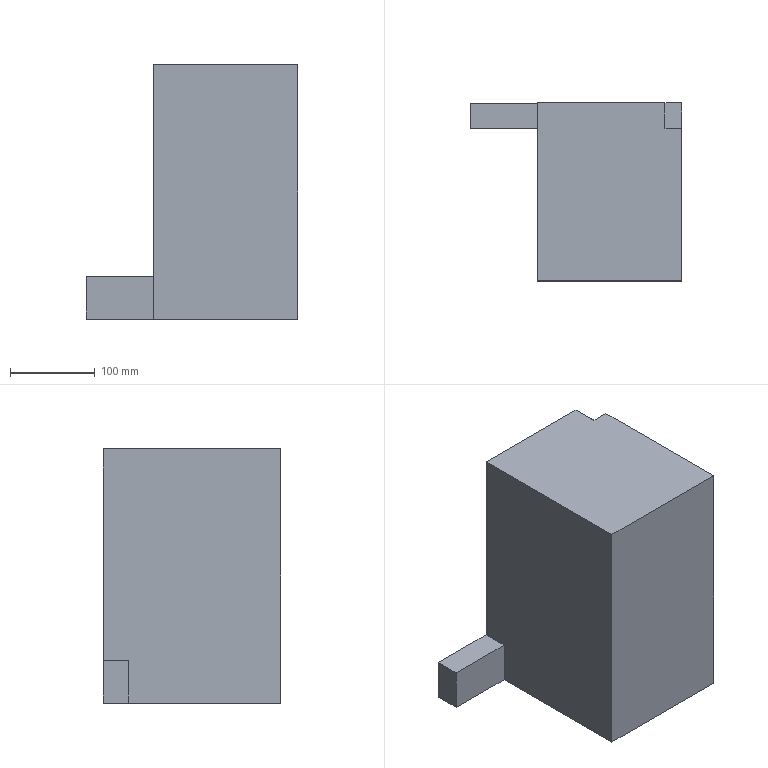Component | SolidWorks | -3[2]-1 | 1 solid | 14 faces | box 250 x 210 x 300 mm | volume 10806823 mm3 | plane 12 | cylinder 2 | commonest cylinder face diameters 27 x2
STEP:
#1=CARTESIAN_POINT('',(19.685,-89.764,-4.39));
#2=VERTEX_POINT('',#1);
#3=CARTESIAN_POINT('',(19.685,-89.764,-5.453));
#4=VERTEX_POINT('',#3);
#5=CARTESIAN_POINT('',(19.685,-89.764,-4.921));
#6=DIRECTION('',(0.,-1.,0.));
#7=DIRECTION('',(0.,0.,1.));
#8=AXIS2_PLACEMENT_3D('',#5,#6,#7);
#9=CIRCLE('',#8,0.5315);
#10=EDGE_CURVE('',#2,#4,#9,.T.);
#11=ORIENTED_EDGE('',*,*,#10,.T.);
#12=CARTESIAN_POINT('',(19.685,-88.583,-5.453));
#13=VERTEX_POINT('',#12);
#14=CARTESIAN_POINT('',(19.685,-89.764,-5.453));
#15=DIRECTION('',(0.,1.,0.));
#16=VECTOR('',#15,39.37);
#17=LINE('',#14,#16);
#18=EDGE_CURVE('',#4,#13,#17,.T.);
#19=ORIENTED_EDGE('',*,*,#18,.T.);
#20=CARTESIAN_POINT('',(19.685,-88.583,-4.39));
#21=VERTEX_POINT('',#20);
#22=CARTESIAN_POINT('',(19.685,-88.583,-4.921));
#23=DIRECTION('',(0.,-1.,0.));
#24=DIRECTION('',(0.,0.,1.));
#25=AXIS2_PLACEMENT_3D('',#22,#23,#24);
#26=CIRCLE('',#25,0.5315);
#27=EDGE_CURVE('',#21,#13,#26,.T.);
#28=ORIENTED_EDGE('',*,*,#27,.F.);
#29=CARTESIAN_POINT('',(19.685,-89.764,-4.39));
#30=DIRECTION('',(0.,1.,0.));
#31=VECTOR('',#30,39.37);
#32=LINE('',#29,#31);
#33=EDGE_CURVE('',#2,#21,#32,.T.);
#34=ORIENTED_EDGE('',*,*,#33,.F.);
#35=EDGE_LOOP('',(#11,#19,#28,#34));
#36=FACE_OUTER_BOUND('',#35,.T.);
#37=CARTESIAN_POINT('',(19.685,-89.764,-4.921));
#38=DIRECTION('',(0.,1.,0.));
#39=DIRECTION('',(0.,0.,-1.));
#40=AXIS2_PLACEMENT_3D('',#37,#38,#39);
#41=CYLINDRICAL_SURFACE('',#40,0.5315);
#42=ADVANCED_FACE('',(#36),#41,.F.);
#43=CARTESIAN_POINT('',(14.961,-89.764,-6.89));
#44=VERTEX_POINT('',#43);
#45=CARTESIAN_POINT('',(14.961,-89.764,-8.858));
#46=VERTEX_POINT('',#45);
#47=CARTESIAN_POINT('',(14.961,-89.764,2.953));
#48=DIRECTION('',(0.,0.,-1.));
#49=VECTOR('',#48,39.37);
#50=LINE('',#47,#49);
#51=EDGE_CURVE('',#44,#46,#50,.T.);
#52=ORIENTED_EDGE('',*,*,#51,.F.);
#53=CARTESIAN_POINT('',(11.811,-89.764,-6.89));
#54=VERTEX_POINT('',#53);
#55=CARTESIAN_POINT('',(14.961,-89.764,-6.89));
#56=DIRECTION('',(-1.,0.,0.));
#57=VECTOR('',#56,39.37);
#58=LINE('',#55,#57);
#59=EDGE_CURVE('',#44,#54,#58,.T.);
#60=ORIENTED_EDGE('',*,*,#59,.T.);
#61=CARTESIAN_POINT('',(11.811,-89.764,-8.858));
#62=VERTEX_POINT('',#61);
#63=CARTESIAN_POINT('',(11.811,-89.764,-6.89));
#64=DIRECTION('',(0.,0.,-1.));
#65=VECTOR('',#64,39.37);
#66=LINE('',#63,#65);
#67=EDGE_CURVE('',#54,#62,#66,.T.);
#68=ORIENTED_EDGE('',*,*,#67,.T.);
#69=CARTESIAN_POINT('',(11.811,-89.764,-8.858));
#70=DIRECTION('',(1.,0.,0.));
#71=VECTOR('',#70,39.37);
#72=LINE('',#69,#71);
#73=EDGE_CURVE('',#62,#46,#72,.T.);
#74=ORIENTED_EDGE('',*,*,#73,.T.);
#75=EDGE_LOOP('',(#52,#60,#68,#74));
#76=FACE_OUTER_BOUND('',#75,.T.);
#77=CARTESIAN_POINT('',(11.811,-89.764,-8.858));
#78=DIRECTION('',(0.,-1.,0.));
#79=DIRECTION('',(0.,0.,1.));
#80=AXIS2_PLACEMENT_3D('',#77,#78,#79);
#81=PLANE('',#80);
#82=ADVANCED_FACE('',(#76),#81,.T.);
#83=CARTESIAN_POINT('',(11.811,-88.583,-6.89));
#84=VERTEX_POINT('',#83);
#85=CARTESIAN_POINT('',(11.811,-88.583,-8.858));
#86=VERTEX_POINT('',#85);
#87=CARTESIAN_POINT('',(11.811,-88.583,-6.89));
#88=DIRECTION('',(0.,0.,-1.));
#89=VECTOR('',#88,39.37);
#90=LINE('',#87,#89);
#91=EDGE_CURVE('',#84,#86,#90,.T.);
#92=ORIENTED_EDGE('',*,*,#91,.F.);
#93=CARTESIAN_POINT('',(14.961,-88.583,-6.89));
#94=VERTEX_POINT('',#93);
#95=CARTESIAN_POINT('',(14.961,-88.583,-6.89));
#96=DIRECTION('',(-1.,0.,0.));
#97=VECTOR('',#96,39.37);
#98=LINE('',#95,#97);
#99=EDGE_CURVE('',#94,#84,#98,.T.);
#100=ORIENTED_EDGE('',*,*,#99,.F.);
#101=CARTESIAN_POINT('',(14.961,-88.583,2.953));
#102=VERTEX_POINT('',#101);
#103=CARTESIAN_POINT('',(14.961,-88.583,2.953));
#104=DIRECTION('',(-0.,0.,-1.));
#105=VECTOR('',#104,39.37);
#106=LINE('',#103,#105);
#107=EDGE_CURVE('',#102,#94,#106,.T.);
#108=ORIENTED_EDGE('',*,*,#107,.F.);
#109=CARTESIAN_POINT('',(20.866,-88.583,2.953));
#110=VERTEX_POINT('',#109);
#111=CARTESIAN_POINT('',(20.866,-88.583,2.953));
#112=DIRECTION('',(-1.,0.,0.));
#113=VECTOR('',#112,39.37);
#114=LINE('',#111,#113);
#115=EDGE_CURVE('',#110,#102,#114,.T.);
#116=ORIENTED_EDGE('',*,*,#115,.F.);
#117=CARTESIAN_POINT('',(21.654,-88.583,2.165));
#118=VERTEX_POINT('',#117);
#119=CARTESIAN_POINT('',(21.654,-88.583,2.165));
#120=DIRECTION('',(-0.7071,0.,0.7071));
#121=VECTOR('',#120,39.37);
#122=LINE('',#119,#121);
#123=EDGE_CURVE('',#118,#110,#122,.T.);
#124=ORIENTED_EDGE('',*,*,#123,.F.);
#125=CARTESIAN_POINT('',(21.654,-88.583,-8.858));
#126=VERTEX_POINT('',#125);
#127=CARTESIAN_POINT('',(21.654,-88.583,-8.858));
#128=DIRECTION('',(0.,0.,1.));
#129=VECTOR('',#128,39.37);
#130=LINE('',#127,#129);
#131=EDGE_CURVE('',#126,#118,#130,.T.);
#132=ORIENTED_EDGE('',*,*,#131,.F.);
#133=CARTESIAN_POINT('',(11.811,-88.583,-8.858));
#134=DIRECTION('',(1.,0.,0.));
#135=VECTOR('',#134,39.37);
#136=LINE('',#133,#135);
#137=EDGE_CURVE('',#86,#126,#136,.T.);
#138=ORIENTED_EDGE('',*,*,#137,.F.);
#139=EDGE_LOOP('',(#92,#100,#108,#116,#124,#132,#138));
#140=FACE_OUTER_BOUND('',#139,.T.);
#141=ORIENTED_EDGE('',*,*,#27,.T.);
#142=CARTESIAN_POINT('',(19.685,-88.583,-4.921));
#143=DIRECTION('',(0.,-1.,0.));
#144=DIRECTION('',(0.,0.,1.));
#145=AXIS2_PLACEMENT_3D('',#142,#143,#144);
#146=CIRCLE('',#145,0.5315);
#147=EDGE_CURVE('',#13,#21,#146,.T.);
#148=ORIENTED_EDGE('',*,*,#147,.T.);
#149=EDGE_LOOP('',(#141,#148));
#150=FACE_BOUND('',#149,.T.);
#151=CARTESIAN_POINT('',(11.811,-88.583,-8.858));
#152=DIRECTION('',(0.,-1.,0.));
#153=DIRECTION('',(0.,0.,1.));
#154=AXIS2_PLACEMENT_3D('',#151,#152,#153);
#155=PLANE('',#154);
#156=ADVANCED_FACE('',(#140,#150),#155,.F.);
#157=ORIENTED_EDGE('',*,*,#91,.T.);
#158=CARTESIAN_POINT('',(11.811,-89.764,-8.858));
#159=DIRECTION('',(0.,1.,0.));
#160=VECTOR('',#159,39.37);
#161=LINE('',#158,#160);
#162=EDGE_CURVE('',#62,#86,#161,.T.);
#163=ORIENTED_EDGE('',*,*,#162,.F.);
#164=ORIENTED_EDGE('',*,*,#67,.F.);
#165=CARTESIAN_POINT('',(11.811,-89.764,-6.89));
#166=DIRECTION('',(0.,1.,0.));
#167=VECTOR('',#166,39.37);
#168=LINE('',#165,#167);
#169=EDGE_CURVE('',#54,#84,#168,.T.);
#170=ORIENTED_EDGE('',*,*,#169,.T.);
#171=EDGE_LOOP('',(#157,#163,#164,#170));
#172=FACE_OUTER_BOUND('',#171,.T.);
#173=CARTESIAN_POINT('',(11.811,-89.764,-6.89));
#174=DIRECTION('',(1.,0.,0.));
#175=DIRECTION('',(0.,0.,1.));
#176=AXIS2_PLACEMENT_3D('',#173,#174,#175);
#177=PLANE('',#176);
#178=ADVANCED_FACE('',(#172),#177,.F.);
#179=ORIENTED_EDGE('',*,*,#137,.T.);
#180=CARTESIAN_POINT('',(21.654,-96.85,-8.858));
#181=VERTEX_POINT('',#180);
#182=CARTESIAN_POINT('',(21.654,-89.764,-8.858));
#183=DIRECTION('',(0.,1.,0.));
#184=VECTOR('',#183,39.37);
#185=LINE('',#182,#184);
#186=EDGE_CURVE('',#181,#126,#185,.T.);
#187=ORIENTED_EDGE('',*,*,#186,.F.);
#188=CARTESIAN_POINT('',(14.961,-96.85,-8.858));
#189=VERTEX_POINT('',#188);
#190=CARTESIAN_POINT('',(14.961,-96.85,-8.858));
#191=DIRECTION('',(1.,0.,0.));
#192=VECTOR('',#191,39.37);
#193=LINE('',#190,#192);
#194=EDGE_CURVE('',#189,#181,#193,.T.);
#195=ORIENTED_EDGE('',*,*,#194,.F.);
#196=CARTESIAN_POINT('',(14.961,-96.85,-8.858));
#197=DIRECTION('',(0.,1.,0.));
#198=VECTOR('',#197,39.37);
#199=LINE('',#196,#198);
#200=EDGE_CURVE('',#189,#46,#199,.T.);
#201=ORIENTED_EDGE('',*,*,#200,.T.);
#202=ORIENTED_EDGE('',*,*,#73,.F.);
#203=ORIENTED_EDGE('',*,*,#162,.T.);
#204=EDGE_LOOP('',(#179,#187,#195,#201,#202,#203));
#205=FACE_OUTER_BOUND('',#204,.T.);
#206=CARTESIAN_POINT('',(11.811,-89.764,-8.858));
#207=DIRECTION('',(0.,0.,1.));
#208=DIRECTION('',(-1.,0.,0.));
#209=AXIS2_PLACEMENT_3D('',#206,#207,#208);
#210=PLANE('',#209);
#211=ADVANCED_FACE('',(#205),#210,.F.);
#212=ORIENTED_EDGE('',*,*,#131,.T.);
#213=CARTESIAN_POINT('',(21.654,-89.764,2.165));
#214=VERTEX_POINT('',#213);
#215=CARTESIAN_POINT('',(21.654,-89.764,2.165));
#216=DIRECTION('',(0.,1.,0.));
#217=VECTOR('',#216,39.37);
#218=LINE('',#215,#217);
#219=EDGE_CURVE('',#214,#118,#218,.T.);
#220=ORIENTED_EDGE('',*,*,#219,.F.);
#221=CARTESIAN_POINT('',(21.654,-89.764,2.953));
#222=VERTEX_POINT('',#221);
#223=CARTESIAN_POINT('',(21.654,-89.764,2.953));
#224=DIRECTION('',(0.,0.,1.));
#225=VECTOR('',#224,39.37);
#226=LINE('',#223,#225);
#227=EDGE_CURVE('',#214,#222,#226,.T.);
#228=ORIENTED_EDGE('',*,*,#227,.T.);
#229=CARTESIAN_POINT('',(21.654,-96.85,2.953));
#230=VERTEX_POINT('',#229);
#231=CARTESIAN_POINT('',(21.654,-96.85,2.953));
#232=DIRECTION('',(0.,1.,0.));
#233=VECTOR('',#232,39.37);
#234=LINE('',#231,#233);
#235=EDGE_CURVE('',#230,#222,#234,.T.);
#236=ORIENTED_EDGE('',*,*,#235,.F.);
#237=CARTESIAN_POINT('',(21.654,-96.85,2.953));
#238=DIRECTION('',(0.,0.,1.));
#239=VECTOR('',#238,39.37);
#240=LINE('',#237,#239);
#241=EDGE_CURVE('',#181,#230,#240,.T.);
#242=ORIENTED_EDGE('',*,*,#241,.F.);
#243=ORIENTED_EDGE('',*,*,#186,.T.);
#244=EDGE_LOOP('',(#212,#220,#228,#236,#242,#243));
#245=FACE_OUTER_BOUND('',#244,.T.);
#246=CARTESIAN_POINT('',(21.654,-89.764,-8.858));
#247=DIRECTION('',(-1.,0.,0.));
#248=DIRECTION('',(0.,0.,-1.));
#249=AXIS2_PLACEMENT_3D('',#246,#247,#248);
#250=PLANE('',#249);
#251=ADVANCED_FACE('',(#245),#250,.F.);
#252=ORIENTED_EDGE('',*,*,#123,.T.);
#253=CARTESIAN_POINT('',(20.866,-89.764,2.953));
#254=VERTEX_POINT('',#253);
#255=CARTESIAN_POINT('',(20.866,-89.764,2.953));
#256=DIRECTION('',(0.,1.,0.));
#257=VECTOR('',#256,39.37);
#258=LINE('',#255,#257);
#259=EDGE_CURVE('',#254,#110,#258,.T.);
#260=ORIENTED_EDGE('',*,*,#259,.F.);
#261=CARTESIAN_POINT('',(21.654,-89.764,2.165));
#262=DIRECTION('',(-0.7071,0.,0.7071));
#263=VECTOR('',#262,39.37);
#264=LINE('',#261,#263);
#265=EDGE_CURVE('',#214,#254,#264,.T.);
#266=ORIENTED_EDGE('',*,*,#265,.F.);
#267=ORIENTED_EDGE('',*,*,#219,.T.);
#268=EDGE_LOOP('',(#252,#260,#266,#267));
#269=FACE_OUTER_BOUND('',#268,.T.);
#270=CARTESIAN_POINT('',(21.654,-89.764,2.165));
#271=DIRECTION('',(-0.7071,0.,-0.7071));
#272=DIRECTION('',(0.7071,0.,-0.7071));
#273=AXIS2_PLACEMENT_3D('',#270,#271,#272);
#274=PLANE('',#273);
#275=ADVANCED_FACE('',(#269),#274,.F.);
#276=ORIENTED_EDGE('',*,*,#115,.T.);
#277=CARTESIAN_POINT('',(14.961,-96.85,2.953));
#278=VERTEX_POINT('',#277);
#279=CARTESIAN_POINT('',(14.961,-89.764,2.953));
#280=DIRECTION('',(0.,1.,0.));
#281=VECTOR('',#280,39.37);
#282=LINE('',#279,#281);
#283=EDGE_CURVE('',#278,#102,#282,.T.);
#284=ORIENTED_EDGE('',*,*,#283,.F.);
#285=CARTESIAN_POINT('',(14.961,-96.85,2.953));
#286=DIRECTION('',(-1.,0.,0.));
#287=VECTOR('',#286,39.37);
#288=LINE('',#285,#287);
#289=EDGE_CURVE('',#230,#278,#288,.T.);
#290=ORIENTED_EDGE('',*,*,#289,.F.);
#291=ORIENTED_EDGE('',*,*,#235,.T.);
#292=CARTESIAN_POINT('',(14.961,-89.764,2.953));
#293=DIRECTION('',(-1.,0.,0.));
#294=VECTOR('',#293,39.37);
#295=LINE('',#292,#294);
#296=EDGE_CURVE('',#222,#254,#295,.T.);
#297=ORIENTED_EDGE('',*,*,#296,.T.);
#298=ORIENTED_EDGE('',*,*,#259,.T.);
#299=EDGE_LOOP('',(#276,#284,#290,#291,#297,#298));
#300=FACE_OUTER_BOUND('',#299,.T.);
#301=CARTESIAN_POINT('',(20.866,-89.764,2.953));
#302=DIRECTION('',(0.,0.,-1.));
#303=DIRECTION('',(1.,0.,0.));
#304=AXIS2_PLACEMENT_3D('',#301,#302,#303);
#305=PLANE('',#304);
#306=ADVANCED_FACE('',(#300),#305,.F.);
#307=ORIENTED_EDGE('',*,*,#107,.T.);
#308=CARTESIAN_POINT('',(14.961,-89.764,-6.89));
#309=DIRECTION('',(0.,1.,0.));
#310=VECTOR('',#309,39.37);
#311=LINE('',#308,#310);
#312=EDGE_CURVE('',#44,#94,#311,.T.);
#313=ORIENTED_EDGE('',*,*,#312,.F.);
#314=ORIENTED_EDGE('',*,*,#51,.T.);
#315=ORIENTED_EDGE('',*,*,#200,.F.);
#316=CARTESIAN_POINT('',(14.961,-96.85,2.953));
#317=DIRECTION('',(0.,0.,-1.));
#318=VECTOR('',#317,39.37);
#319=LINE('',#316,#318);
#320=EDGE_CURVE('',#278,#189,#319,.T.);
#321=ORIENTED_EDGE('',*,*,#320,.F.);
#322=ORIENTED_EDGE('',*,*,#283,.T.);
#323=EDGE_LOOP('',(#307,#313,#314,#315,#321,#322));
#324=FACE_OUTER_BOUND('',#323,.T.);
#325=CARTESIAN_POINT('',(14.961,-89.764,2.953));
#326=DIRECTION('',(1.,0.,-0.));
#327=DIRECTION('',(0.,0.,1.));
#328=AXIS2_PLACEMENT_3D('',#325,#326,#327);
#329=PLANE('',#328);
#330=ADVANCED_FACE('',(#324),#329,.F.);
#331=ORIENTED_EDGE('',*,*,#99,.T.);
#332=ORIENTED_EDGE('',*,*,#169,.F.);
#333=ORIENTED_EDGE('',*,*,#59,.F.);
#334=ORIENTED_EDGE('',*,*,#312,.T.);
#335=EDGE_LOOP('',(#331,#332,#333,#334));
#336=FACE_OUTER_BOUND('',#335,.T.);
#337=CARTESIAN_POINT('',(14.961,-89.764,-6.89));
#338=DIRECTION('',(0.,0.,-1.));
#339=DIRECTION('',(1.,0.,0.));
#340=AXIS2_PLACEMENT_3D('',#337,#338,#339);
#341=PLANE('',#340);
#342=ADVANCED_FACE('',(#336),#341,.F.);
#343=ORIENTED_EDGE('',*,*,#18,.F.);
#344=CARTESIAN_POINT('',(19.685,-89.764,-4.921));
#345=DIRECTION('',(0.,-1.,0.));
#346=DIRECTION('',(0.,0.,1.));
#347=AXIS2_PLACEMENT_3D('',#344,#345,#346);
#348=CIRCLE('',#347,0.5315);
#349=EDGE_CURVE('',#4,#2,#348,.T.);
#350=ORIENTED_EDGE('',*,*,#349,.T.);
#351=ORIENTED_EDGE('',*,*,#33,.T.);
#352=ORIENTED_EDGE('',*,*,#147,.F.);
#353=EDGE_LOOP('',(#343,#350,#351,#352));
#354=FACE_OUTER_BOUND('',#353,.T.);
#355=CARTESIAN_POINT('',(19.685,-89.764,-4.921));
#356=DIRECTION('',(0.,1.,0.));
#357=DIRECTION('',(0.,0.,-1.));
#358=AXIS2_PLACEMENT_3D('',#355,#356,#357);
#359=CYLINDRICAL_SURFACE('',#358,0.5315);
#360=ADVANCED_FACE('',(#354),#359,.F.);
#361=ORIENTED_EDGE('',*,*,#320,.T.);
#362=ORIENTED_EDGE('',*,*,#194,.T.);
#363=ORIENTED_EDGE('',*,*,#241,.T.);
#364=ORIENTED_EDGE('',*,*,#289,.T.);
#365=EDGE_LOOP('',(#361,#362,#363,#364));
#366=FACE_OUTER_BOUND('',#365,.T.);
#367=CARTESIAN_POINT('',(0.,-96.85,0.));
#368=DIRECTION('',(0.,-1.,0.));
#369=DIRECTION('',(0.,0.,1.));
#370=AXIS2_PLACEMENT_3D('',#367,#368,#369);
#371=PLANE('',#370);
#372=ADVANCED_FACE('',(#366),#371,.T.);
#373=ORIENTED_EDGE('',*,*,#227,.F.);
#374=ORIENTED_EDGE('',*,*,#265,.T.);
#375=ORIENTED_EDGE('',*,*,#296,.F.);
#376=EDGE_LOOP('',(#373,#374,#375));
#377=FACE_OUTER_BOUND('',#376,.T.);
#378=CARTESIAN_POINT('',(0.,-89.764,0.));
#379=DIRECTION('',(0.,-1.,0.));
#380=DIRECTION('',(0.,0.,1.));
#381=AXIS2_PLACEMENT_3D('',#378,#379,#380);
#382=PLANE('',#381);
#383=ADVANCED_FACE('',(#377),#382,.F.);
#384=ORIENTED_EDGE('',*,*,#10,.F.);
#385=ORIENTED_EDGE('',*,*,#349,.F.);
#386=EDGE_LOOP('',(#384,#385));
#387=FACE_OUTER_BOUND('',#386,.T.);
#388=CARTESIAN_POINT('',(0.,-89.764,0.));
#389=DIRECTION('',(0.,-1.,0.));
#390=DIRECTION('',(0.,0.,1.));
#391=AXIS2_PLACEMENT_3D('',#388,#389,#390);
#392=PLANE('',#391);
#393=ADVANCED_FACE('',(#387),#392,.F.);
#394=CLOSED_SHELL('',(#42,#82,#156,#178,#211,#251,#275,#306,#330,#342,#360,#372,#383,#393));
#395=MANIFOLD_SOLID_BREP('',#394);
#396=CARTESIAN_POINT('',(0.,0.,0.));
#397=DIRECTION('',(0.,0.,1.));
#398=DIRECTION('',(1.,0.,0.));
#399=AXIS2_PLACEMENT_3D('',#396,#397,#398);
#400=(LENGTH_UNIT()NAMED_UNIT(*)SI_UNIT($,.METRE.));
#401=LENGTH_MEASURE_WITH_UNIT(LENGTH_MEASURE(0.0254),#400);
#402=DIMENSIONAL_EXPONENTS(1.,0.,0.,0.,0.,0.,0.);
#403=(CONVERSION_BASED_UNIT('',#401)LENGTH_UNIT()NAMED_UNIT(#402));
#404=UNCERTAINTY_MEASURE_WITH_UNIT(LENGTH_MEASURE(0.00001),#403,'','');
#405=(NAMED_UNIT(*)PLANE_ANGLE_UNIT()SI_UNIT($,.RADIAN.));
#406=(NAMED_UNIT(*)SI_UNIT($,.STERADIAN.)SOLID_ANGLE_UNIT());
#407=(GEOMETRIC_REPRESENTATION_CONTEXT(3)GLOBAL_UNCERTAINTY_ASSIGNED_CONTEXT((#404))GLOBAL_UNIT_ASSIGNED_CONTEXT((#403,#405,#406))REPRESENTATION_CONTEXT('',''));
#408=ADVANCED_BREP_SHAPE_REPRESENTATION('',(#395,#399),#407);
#409=COLOUR_RGB('',0.7922,0.8196,0.9333);
#410=FILL_AREA_STYLE_COLOUR('',#409);
#411=FILL_AREA_STYLE('',(#410));
#412=SURFACE_STYLE_FILL_AREA(#411);
#413=SURFACE_SIDE_STYLE('',(#412));
#414=SURFACE_STYLE_USAGE(.BOTH.,#413);
#415=PRESENTATION_STYLE_ASSIGNMENT((#414));
#416=STYLED_ITEM('',(#415),#395);
#417=PRESENTATION_LAYER_ASSIGNMENT('','',(#416));
#418=(LENGTH_UNIT()NAMED_UNIT(*)SI_UNIT($,.METRE.));
#419=LENGTH_MEASURE_WITH_UNIT(LENGTH_MEASURE(0.0254),#418);
#420=DIMENSIONAL_EXPONENTS(1.,0.,0.,0.,0.,0.,0.);
#421=(CONVERSION_BASED_UNIT('',#419)LENGTH_UNIT()NAMED_UNIT(#420));
#422=UNCERTAINTY_MEASURE_WITH_UNIT(LENGTH_MEASURE(0.00001),#421,'','');
#423=(NAMED_UNIT(*)PLANE_ANGLE_UNIT()SI_UNIT($,.RADIAN.));
#424=(NAMED_UNIT(*)SI_UNIT($,.STERADIAN.)SOLID_ANGLE_UNIT());
#425=(GEOMETRIC_REPRESENTATION_CONTEXT(3)GLOBAL_UNCERTAINTY_ASSIGNED_CONTEXT((#422))GLOBAL_UNIT_ASSIGNED_CONTEXT((#421,#423,#424))REPRESENTATION_CONTEXT('',''));
#426=MECHANICAL_DESIGN_GEOMETRIC_PRESENTATION_REPRESENTATION('',(#416),#425);